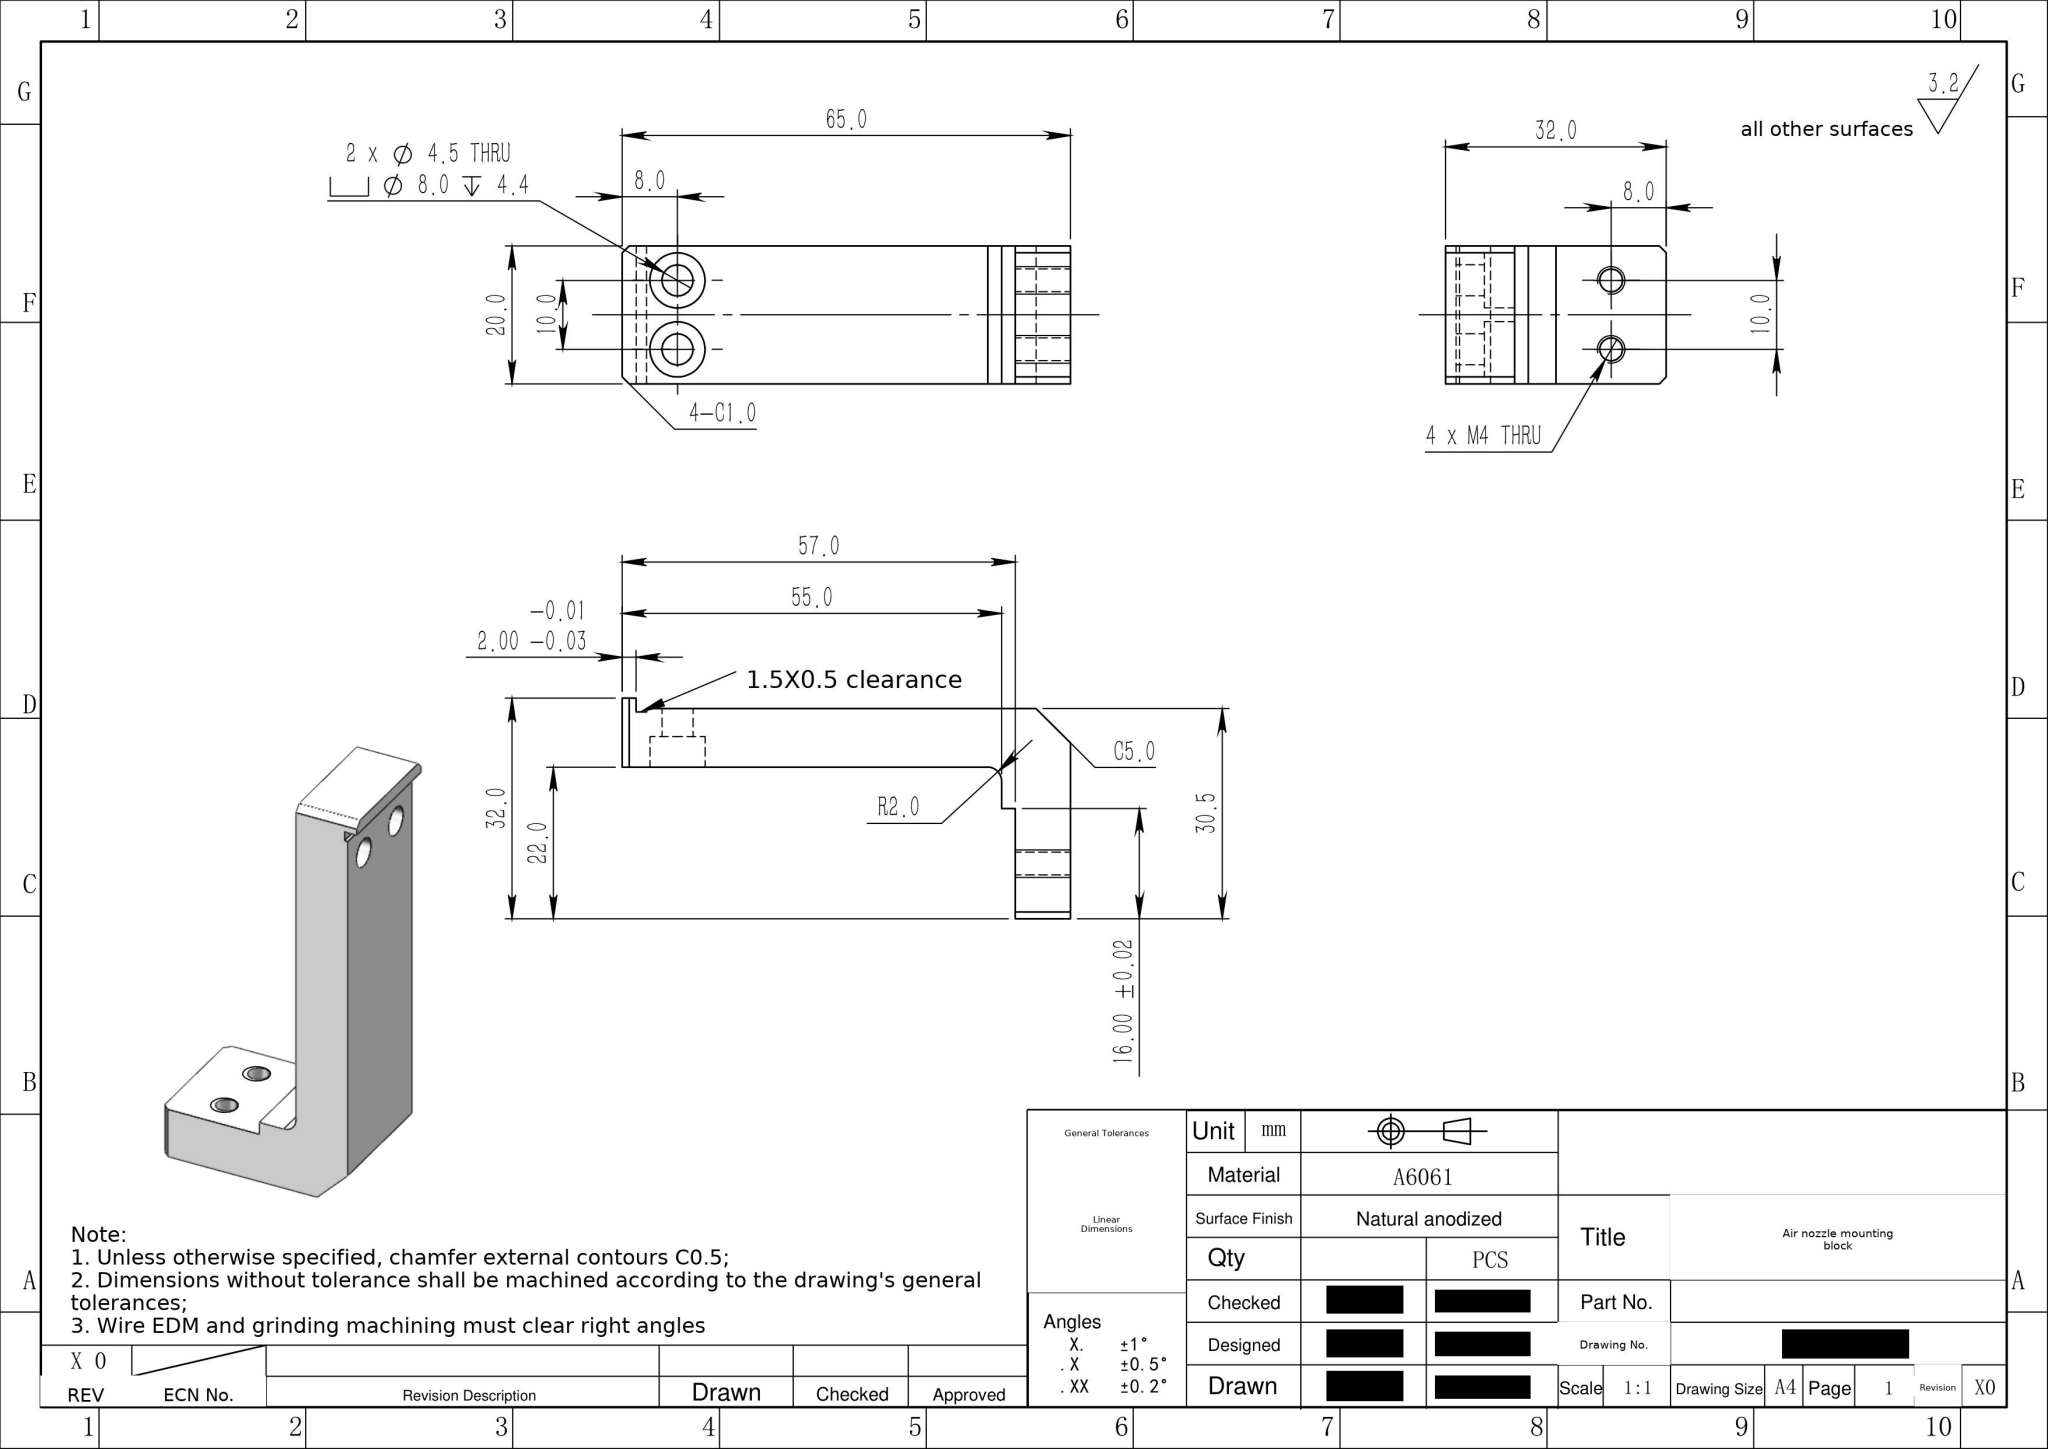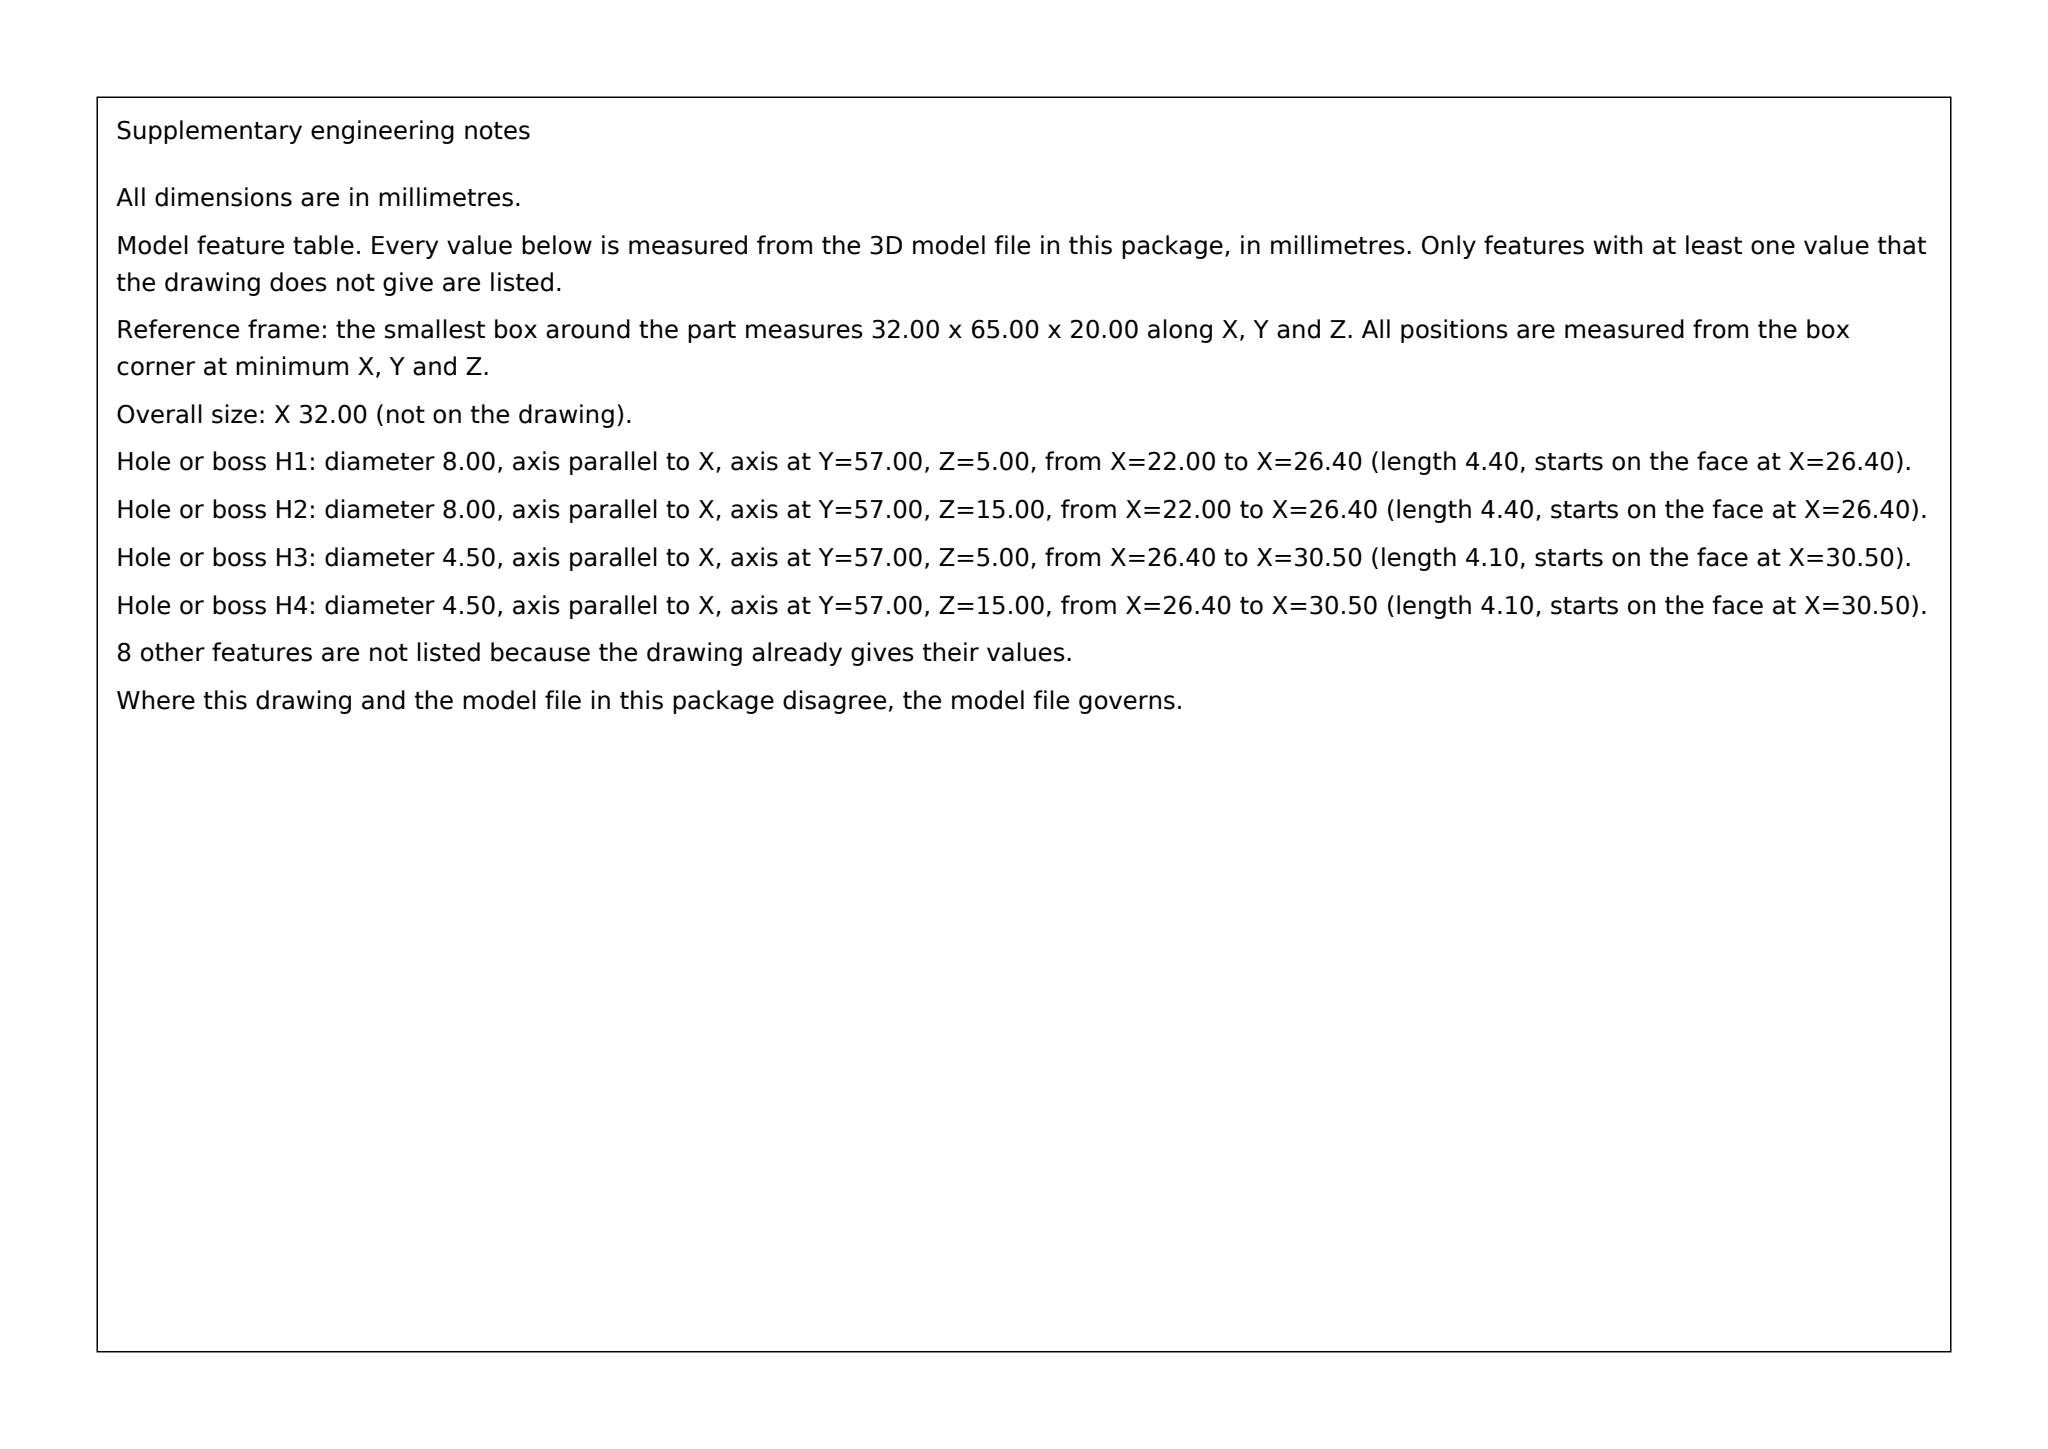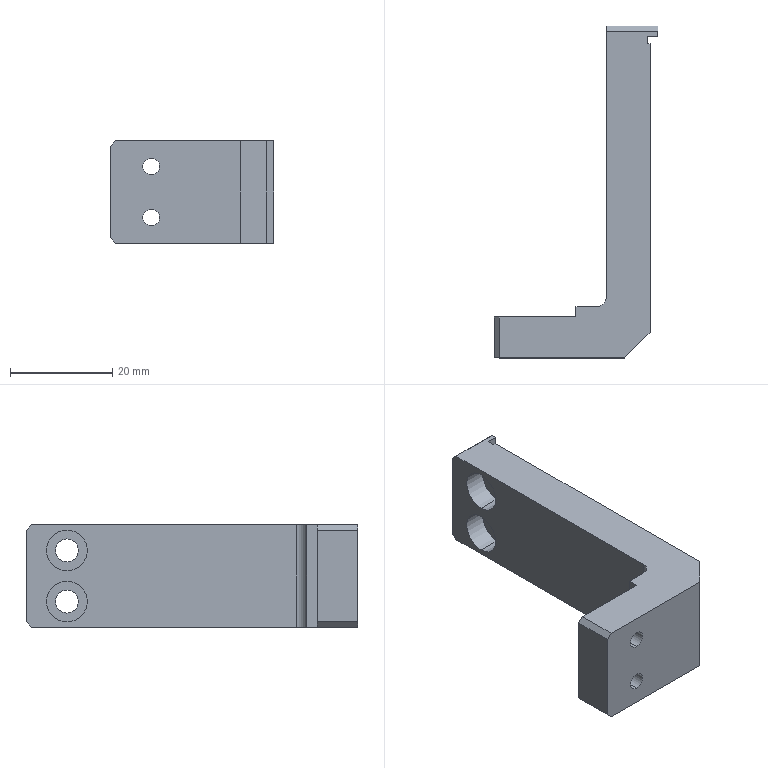Part | SolidWorks | mm | material A6061 | 1 solid | 34 faces | box 32 x 65 x 20 mm | volume 13895 mm3 | plane 21 | cylinder 13 | commonest cylinder face diameters 3.3 x4 8 x4 4.5 x4 4 x1
build123d program:
from build123d import *

# Parameters (mm, degrees)
SKETCH1_W                                       = 32
SKETCH1_H                                       = 65
BOSS_EXTRUDE1_DEPTH                             = 120
SKETCH2_W                                       = 22
SKETCH2_H                                       = 55
CUT_EXTRUDE1_DEPTH                              = 126.349
SKETCH3_W                                       = 1.5
SKETCH3_H                                       = 63
CUT_EXTRUDE2_DEPTH                              = 126.349
SKETCH4_W                                       = 0.5
SKETCH4_H                                       = 1.5
CUT_EXTRUDE3_DEPTH                              = 126.349
SKETCH5_W                                       = 80
SKETCH5_H                                       = 50
CUT_EXTRUDE4_DEPTH                              = 129.375
SKETCH9_W                                       = 16
SKETCH9_H                                       = 2
CUT_EXTRUDE6_DEPTH                              = 126.349
FILLET1_R                                       = 2
M4_HEX_SOCKET_HEAD_CAP_SCREW_CBORE1_D           = 4.5
M4_HEX_SOCKET_HEAD_CAP_SCREW_CBORE1_CBORE_D     = 8
M4_HEX_SOCKET_HEAD_CAP_SCREW_CBORE1_CBORE_DEPTH = 4.4
SKETCH12_W                                      = 1.5
SKETCH12_H                                      = 100
CUT_EXTRUDE7_DEPTH                              = 137.473
M4_TAPPED_HOLE1_D                               = 3.3
SKETCH15_W                                      = 100
SKETCH15_H                                      = 65
CUT_EXTRUDE9_DEPTH                              = 129.375
CHAMFER1_SIZE                                   = 5
CHAMFER2_SIZE                                   = 1


with BuildPart() as part:
    # Sketch1 → Boss-Extrude1 (new body)
    with BuildSketch(Plane.XY):
        Rectangle(SKETCH1_W, SKETCH1_H)
    extrude(amount=-BOSS_EXTRUDE1_DEPTH)

    # Sketch2 → Cut-Extrude1 (cut, through all)
    with BuildSketch(Plane.XY):
        with Locations((-5, 5)):
            Rectangle(SKETCH2_W, SKETCH2_H)
    extrude(amount=-CUT_EXTRUDE1_DEPTH, mode=Mode.SUBTRACT)

    # Sketch3 → Cut-Extrude2 (cut, through all)
    with BuildSketch(Plane.XY):
        with Locations((15.25, -1)):
            Rectangle(SKETCH3_W, SKETCH3_H)
    extrude(amount=-CUT_EXTRUDE2_DEPTH, mode=Mode.SUBTRACT)

    # Sketch4 → Cut-Extrude3 (cut, through all)
    with BuildSketch(Plane.XY):
        with Locations((14.25, 29.75)):
            Rectangle(SKETCH4_W, SKETCH4_H)
    extrude(amount=-CUT_EXTRUDE3_DEPTH, mode=Mode.SUBTRACT)

    # Sketch5 → Cut-Extrude4 (cut, through all)
    with BuildSketch(Plane.ZY.offset(16)):
        with Locations((-60, -7.5)):
            Rectangle(SKETCH5_W, SKETCH5_H)
    extrude(amount=-CUT_EXTRUDE4_DEPTH, mode=Mode.SUBTRACT)

    # Sketch9 → Cut-Extrude6 (cut, through all)
    with BuildSketch(Plane.XY):
        with Locations((-8, -23.5)):
            Rectangle(SKETCH9_W, SKETCH9_H)
    extrude(amount=-CUT_EXTRUDE6_DEPTH, mode=Mode.SUBTRACT)

    # Fillet1
    fillet1_edges = [part.edges().sort_by_distance(p)[0] for p in [
        (6, -22.5, -110),
        (6, -22.5, -10),
    ]]
    fillet(fillet1_edges, radius=FILLET1_R)

    # M4 Hex Socket Head Cap Screw CBORE1 (through all)
    with Locations(Plane.ZY.offset(-6)):
        with Locations((-105, 24.5), (-115, 24.5)):
            CounterBoreHole(M4_HEX_SOCKET_HEAD_CAP_SCREW_CBORE1_D / 2, M4_HEX_SOCKET_HEAD_CAP_SCREW_CBORE1_CBORE_D / 2, M4_HEX_SOCKET_HEAD_CAP_SCREW_CBORE1_CBORE_DEPTH)

    # Sketch12 → Cut-Extrude7 (cut, through all)
    with BuildSketch(Plane.XZ.offset(-30.5)):
        with Locations((15.25, -50)):
            Rectangle(SKETCH12_W, SKETCH12_H)
    extrude(amount=-CUT_EXTRUDE7_DEPTH, mode=Mode.SUBTRACT)

    # M4 Tapped Hole1 (through all)
    with Locations(Plane(origin=(0, -24.5, 0), x_dir=(1, 0, 0), z_dir=(0, 1, 0))):
        with Locations((-8, 5), (-8, 115), (-8, 105), (-8, 15)):
            Hole(M4_TAPPED_HOLE1_D / 2)

    # Sketch15 → Cut-Extrude9 (cut, through all)
    with BuildSketch(Plane.ZY.offset(16)):
        with Locations((-50, 0)):
            Rectangle(SKETCH15_W, SKETCH15_H)
    extrude(amount=-CUT_EXTRUDE9_DEPTH, mode=Mode.SUBTRACT)

    # Chamfer1
    chamfer1_edges = [part.edges().sort_by_distance(p)[0] for p in [
        (14.5, -32.5, -110),
    ]]
    chamfer(chamfer1_edges, length=CHAMFER1_SIZE)

    # Chamfer2
    chamfer2_edges = [part.edges().sort_by_distance(p)[0] for p in [
        (11, 32.5, -100),
        (11, 32.5, -120),
        (-16, -28.5, -100),
        (-16, -28.5, -120),
    ]]
    chamfer(chamfer2_edges, length=CHAMFER2_SIZE)


solid = part.part